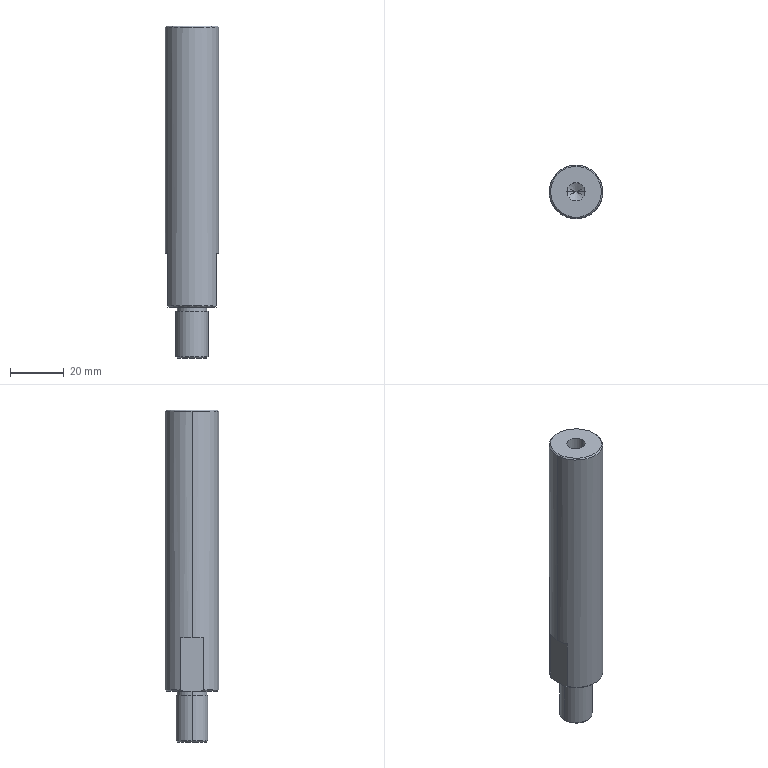Component | SolidWorks | SupportWheelAssembly-1_SupportWheelAxis-1 | 1 solid | 24 faces | box 20 x 20 x 124 mm | volume 34114 mm3 | cylinder 8 | cone 8 | plane 8 | commonest cylinder face diameters 6.8 x2 12 x2 11 x2 20 x2
build123d program:
from build123d import *

# Parameters (mm, degrees)
SKETCH1_R             = 10
BOSS_EXTRUDE1_DEPTH   = 52.5
CHAMFER1_SIZE         = 0.5
SKETCH4_W             = 7.858
SKETCH4_H             = 16.97
SKETCH4_W_2           = 6.894
SKETCH4_H_2           = 20.345
CUT_EXTRUDE1_DEPTH    = 20
SKETCH5_R             = 6
BOSS_EXTRUDE2_DEPTH   = 19
CHAMFER2_SIZE         = 0.5
SKETCH6_R             = 6
SKETCH6_R_2           = 5.5
CUT_EXTRUDE2_DEPTH    = 1.5
M8_TAPPED_HOLE1_D     = 6.8
M8_TAPPED_HOLE1_DEPTH = 19.75
M8_TAPPED_HOLE1_TIP   = 2.043


with BuildPart() as part:
    # Sketch1 → Boss-Extrude1 (new, symmetric)
    with BuildSketch(Plane.XY):
        Circle(SKETCH1_R)
    extrude(amount=BOSS_EXTRUDE1_DEPTH, both=True)

    # Chamfer1
    chamfer1_edges = [part.edges().sort_by_distance(p)[0] for p in [
        (-10, 0, -52.5),
        (-10, 0, 52.5),
    ]]
    chamfer(chamfer1_edges, length=CHAMFER1_SIZE)

    # Sketch4 → Cut-Extrude1 (cut)
    with BuildSketch(Plane(origin=(0, 0, -52.5), x_dir=(-1, 0, 0), z_dir=(0, 0, -1))):
        with Locations((-12.929, 0.3857)):
            Rectangle(SKETCH4_W, SKETCH4_H)
        with Locations((12.447, -0.916)):
            Rectangle(SKETCH4_W_2, SKETCH4_H_2)
    extrude(amount=-CUT_EXTRUDE1_DEPTH, mode=Mode.SUBTRACT)

    # Sketch5 → Boss-Extrude2 (add)
    with BuildSketch(Plane(origin=(0, 0, -52.5), x_dir=(-1, 0, 0), z_dir=(0, 0, -1))):
        with Locations(Location((0, 0, 0), (0, 0, 180))):
            Circle(SKETCH5_R)
    extrude(amount=BOSS_EXTRUDE2_DEPTH)

    # Chamfer2
    chamfer2_edges = [part.edges().sort_by_distance(p)[0] for p in [
        (-6, 0, -71.5),
    ]]
    chamfer(chamfer2_edges, length=CHAMFER2_SIZE)

    # Sketch6 → Cut-Extrude2 (cut)
    with BuildSketch(Plane(origin=(0, 0, -52.5), x_dir=(-1, 0, 0), z_dir=(0, 0, -1))):
        Circle(SKETCH6_R)
        Circle(SKETCH6_R_2, mode=Mode.SUBTRACT)
    extrude(amount=CUT_EXTRUDE2_DEPTH, mode=Mode.SUBTRACT)

    # M8 Tapped Hole1
    with Locations(Plane.XY.offset(52.5)):
        with Locations((0, 0)):
            Hole(M8_TAPPED_HOLE1_D / 2, depth=M8_TAPPED_HOLE1_DEPTH)
            with Locations((0, 0, -(M8_TAPPED_HOLE1_DEPTH + M8_TAPPED_HOLE1_TIP / 2))):  # 118° drill point
                Cone(0, M8_TAPPED_HOLE1_D / 2, M8_TAPPED_HOLE1_TIP, mode=Mode.SUBTRACT)


solid = part.part

# Placed as in the assembly
solid = solid.moved(Location((-187.007, -195.411, 567.5), (0, 0, 0)))
STEP:
#1=COLOUR_RGB('',0.7922,0.8196,0.9333);
#2=FILL_AREA_STYLE_COLOUR('',#1);
#3=FILL_AREA_STYLE('',(#2));
#4=SURFACE_STYLE_FILL_AREA(#3);
#5=SURFACE_SIDE_STYLE('',(#4));
#6=SURFACE_STYLE_USAGE(.BOTH.,#5);
#7=PRESENTATION_STYLE_ASSIGNMENT((#6));
#8=CARTESIAN_POINT('',(-7.496,-7.693,23.632));
#9=VERTEX_POINT('',#8);
#10=CARTESIAN_POINT('',(-7.229,-7.693,23.632));
#11=VERTEX_POINT('',#10);
#12=CARTESIAN_POINT('',(-7.362,-7.693,23.632));
#13=DIRECTION('',(0.,0.,1.));
#14=DIRECTION('',(1.,0.,0.));
#15=AXIS2_PLACEMENT_3D('',#12,#13,#14);
#16=CIRCLE('',#15,0.1339);
#17=EDGE_CURVE('',#9,#11,#16,.T.);
#18=ORIENTED_EDGE('',*,*,#17,.F.);
#19=CARTESIAN_POINT('',(-7.496,-7.693,24.409));
#20=VERTEX_POINT('',#19);
#21=CARTESIAN_POINT('',(-7.496,-7.693,24.409));
#22=DIRECTION('',(0.,0.,1.));
#23=VECTOR('',#22,39.37);
#24=LINE('',#21,#23);
#25=EDGE_CURVE('',#9,#20,#24,.T.);
#26=ORIENTED_EDGE('',*,*,#25,.T.);
#27=CARTESIAN_POINT('',(-7.229,-7.693,24.409));
#28=VERTEX_POINT('',#27);
#29=CARTESIAN_POINT('',(-7.362,-7.693,24.409));
#30=DIRECTION('',(0.,0.,1.));
#31=DIRECTION('',(1.,0.,0.));
#32=AXIS2_PLACEMENT_3D('',#29,#30,#31);
#33=CIRCLE('',#32,0.1339);
#34=EDGE_CURVE('',#20,#28,#33,.T.);
#35=ORIENTED_EDGE('',*,*,#34,.T.);
#36=CARTESIAN_POINT('',(-7.229,-7.693,24.409));
#37=DIRECTION('',(0.,0.,1.));
#38=VECTOR('',#37,39.37);
#39=LINE('',#36,#38);
#40=EDGE_CURVE('',#11,#28,#39,.T.);
#41=ORIENTED_EDGE('',*,*,#40,.F.);
#42=EDGE_LOOP('',(#18,#26,#35,#41));
#43=FACE_OUTER_BOUND('',#42,.T.);
#44=CARTESIAN_POINT('',(-7.362,-7.693,24.409));
#45=DIRECTION('',(0.,0.,1.));
#46=DIRECTION('',(1.,0.,0.));
#47=AXIS2_PLACEMENT_3D('',#44,#45,#46);
#48=CYLINDRICAL_SURFACE('',#47,0.1339);
#49=ADVANCED_FACE('',(#43),#48,.F.);
#50=CARTESIAN_POINT('',(-7.362,-7.693,23.551));
#51=VERTEX_POINT('',#50);
#52=CARTESIAN_POINT('',(-7.229,-7.693,23.632));
#53=DIRECTION('',(0.8572,0.,0.515));
#54=VECTOR('',#53,39.37);
#55=LINE('',#52,#54);
#56=EDGE_CURVE('',#51,#11,#55,.T.);
#57=ORIENTED_EDGE('',*,*,#56,.F.);
#58=CARTESIAN_POINT('',(-7.496,-7.693,23.632));
#59=DIRECTION('',(-0.8572,0.,0.515));
#60=VECTOR('',#59,39.37);
#61=LINE('',#58,#60);
#62=EDGE_CURVE('',#51,#9,#61,.T.);
#63=ORIENTED_EDGE('',*,*,#62,.T.);
#64=ORIENTED_EDGE('',*,*,#17,.T.);
#65=EDGE_LOOP('',(#57,#63,#64));
#66=FACE_OUTER_BOUND('',#65,.T.);
#67=CARTESIAN_POINT('',(-7.362,-7.693,23.632));
#68=DIRECTION('',(0.,0.,1.));
#69=DIRECTION('',(1.,0.,0.));
#70=AXIS2_PLACEMENT_3D('',#67,#68,#69);
#71=CONICAL_SURFACE('',#70,0.1339,1.03);
#72=ADVANCED_FACE('',(#66),#71,.F.);
#73=CARTESIAN_POINT('',(-7.126,-7.693,19.547));
#74=VERTEX_POINT('',#73);
#75=CARTESIAN_POINT('',(-7.599,-7.693,19.547));
#76=VERTEX_POINT('',#75);
#77=CARTESIAN_POINT('',(-7.362,-7.693,19.547));
#78=DIRECTION('',(0.,0.,1.));
#79=DIRECTION('',(-1.,0.,0.));
#80=AXIS2_PLACEMENT_3D('',#77,#78,#79);
#81=CIRCLE('',#80,0.2362);
#82=EDGE_CURVE('',#74,#76,#81,.T.);
#83=ORIENTED_EDGE('',*,*,#82,.T.);
#84=CARTESIAN_POINT('',(-7.599,-7.693,20.217));
#85=VERTEX_POINT('',#84);
#86=CARTESIAN_POINT('',(-7.599,-7.693,19.528));
#87=DIRECTION('',(0.,0.,1.));
#88=VECTOR('',#87,39.37);
#89=LINE('',#86,#88);
#90=EDGE_CURVE('',#76,#85,#89,.T.);
#91=ORIENTED_EDGE('',*,*,#90,.T.);
#92=CARTESIAN_POINT('',(-7.126,-7.693,20.217));
#93=VERTEX_POINT('',#92);
#94=CARTESIAN_POINT('',(-7.362,-7.693,20.217));
#95=DIRECTION('',(0.,0.,-1.));
#96=DIRECTION('',(-1.,0.,0.));
#97=AXIS2_PLACEMENT_3D('',#94,#95,#96);
#98=CIRCLE('',#97,0.2362);
#99=EDGE_CURVE('',#85,#93,#98,.T.);
#100=ORIENTED_EDGE('',*,*,#99,.T.);
#101=CARTESIAN_POINT('',(-7.126,-7.693,19.528));
#102=DIRECTION('',(0.,0.,1.));
#103=VECTOR('',#102,39.37);
#104=LINE('',#101,#103);
#105=EDGE_CURVE('',#74,#93,#104,.T.);
#106=ORIENTED_EDGE('',*,*,#105,.F.);
#107=EDGE_LOOP('',(#83,#91,#100,#106));
#108=FACE_OUTER_BOUND('',#107,.T.);
#109=CARTESIAN_POINT('',(-7.362,-7.693,19.528));
#110=DIRECTION('',(0.,0.,1.));
#111=DIRECTION('',(1.,0.,0.));
#112=AXIS2_PLACEMENT_3D('',#109,#110,#111);
#113=CYLINDRICAL_SURFACE('',#112,0.2362);
#114=ADVANCED_FACE('',(#108),#113,.T.);
#115=CARTESIAN_POINT('',(-7.579,-7.693,19.528));
#116=VERTEX_POINT('',#115);
#117=CARTESIAN_POINT('',(-7.146,-7.693,19.528));
#118=VERTEX_POINT('',#117);
#119=CARTESIAN_POINT('',(-7.362,-7.693,19.528));
#120=DIRECTION('',(0.,0.,-1.));
#121=DIRECTION('',(-1.,0.,0.));
#122=AXIS2_PLACEMENT_3D('',#119,#120,#121);
#123=CIRCLE('',#122,0.2165);
#124=EDGE_CURVE('',#116,#118,#123,.T.);
#125=ORIENTED_EDGE('',*,*,#124,.F.);
#126=CARTESIAN_POINT('',(-7.579,-7.693,19.528));
#127=DIRECTION('',(-0.7071,0.,0.7071));
#128=VECTOR('',#127,39.37);
#129=LINE('',#126,#128);
#130=EDGE_CURVE('',#116,#76,#129,.T.);
#131=ORIENTED_EDGE('',*,*,#130,.T.);
#132=ORIENTED_EDGE('',*,*,#82,.F.);
#133=CARTESIAN_POINT('',(-7.146,-7.693,19.528));
#134=DIRECTION('',(0.7071,0.,0.7071));
#135=VECTOR('',#134,39.37);
#136=LINE('',#133,#135);
#137=EDGE_CURVE('',#118,#74,#136,.T.);
#138=ORIENTED_EDGE('',*,*,#137,.F.);
#139=EDGE_LOOP('',(#125,#131,#132,#138));
#140=FACE_OUTER_BOUND('',#139,.T.);
#141=CARTESIAN_POINT('',(-7.362,-7.693,19.528));
#142=DIRECTION('',(0.,0.,1.));
#143=DIRECTION('',(1.,0.,0.));
#144=AXIS2_PLACEMENT_3D('',#141,#142,#143);
#145=CONICAL_SURFACE('',#144,0.2165,0.7854);
#146=ADVANCED_FACE('',(#140),#145,.T.);
#147=CARTESIAN_POINT('',(-7.579,-7.693,20.217));
#148=VERTEX_POINT('',#147);
#149=CARTESIAN_POINT('',(-7.146,-7.693,20.217));
#150=VERTEX_POINT('',#149);
#151=CARTESIAN_POINT('',(-7.362,-7.693,20.217));
#152=DIRECTION('',(0.,0.,-1.));
#153=DIRECTION('',(-1.,0.,0.));
#154=AXIS2_PLACEMENT_3D('',#151,#152,#153);
#155=CIRCLE('',#154,0.2165);
#156=EDGE_CURVE('',#148,#150,#155,.T.);
#157=ORIENTED_EDGE('',*,*,#156,.F.);
#158=CARTESIAN_POINT('',(-7.579,-7.693,20.276));
#159=VERTEX_POINT('',#158);
#160=CARTESIAN_POINT('',(-7.579,-7.693,20.217));
#161=DIRECTION('',(0.,0.,1.));
#162=VECTOR('',#161,39.37);
#163=LINE('',#160,#162);
#164=EDGE_CURVE('',#148,#159,#163,.T.);
#165=ORIENTED_EDGE('',*,*,#164,.T.);
#166=CARTESIAN_POINT('',(-7.146,-7.693,20.276));
#167=VERTEX_POINT('',#166);
#168=CARTESIAN_POINT('',(-7.362,-7.693,20.276));
#169=DIRECTION('',(0.,0.,-1.));
#170=DIRECTION('',(-1.,0.,0.));
#171=AXIS2_PLACEMENT_3D('',#168,#169,#170);
#172=CIRCLE('',#171,0.2165);
#173=EDGE_CURVE('',#159,#167,#172,.T.);
#174=ORIENTED_EDGE('',*,*,#173,.T.);
#175=CARTESIAN_POINT('',(-7.146,-7.693,20.217));
#176=DIRECTION('',(0.,0.,1.));
#177=VECTOR('',#176,39.37);
#178=LINE('',#175,#177);
#179=EDGE_CURVE('',#150,#167,#178,.T.);
#180=ORIENTED_EDGE('',*,*,#179,.F.);
#181=EDGE_LOOP('',(#157,#165,#174,#180));
#182=FACE_OUTER_BOUND('',#181,.T.);
#183=CARTESIAN_POINT('',(-7.362,-7.693,20.217));
#184=DIRECTION('',(0.,0.,1.));
#185=DIRECTION('',(1.,0.,0.));
#186=AXIS2_PLACEMENT_3D('',#183,#184,#185);
#187=CYLINDRICAL_SURFACE('',#186,0.2165);
#188=ADVANCED_FACE('',(#182),#187,.T.);
#189=CARTESIAN_POINT('',(-6.988,-7.693,24.409));
#190=VERTEX_POINT('',#189);
#191=CARTESIAN_POINT('',(-7.736,-7.693,24.409));
#192=VERTEX_POINT('',#191);
#193=CARTESIAN_POINT('',(-7.362,-7.693,24.409));
#194=DIRECTION('',(0.,0.,1.));
#195=DIRECTION('',(1.,0.,0.));
#196=AXIS2_PLACEMENT_3D('',#193,#194,#195);
#197=CIRCLE('',#196,0.374);
#198=EDGE_CURVE('',#190,#192,#197,.T.);
#199=ORIENTED_EDGE('',*,*,#198,.F.);
#200=CARTESIAN_POINT('',(-6.969,-7.693,24.39));
#201=VERTEX_POINT('',#200);
#202=CARTESIAN_POINT('',(-6.988,-7.693,24.409));
#203=DIRECTION('',(0.7071,0.,-0.7071));
#204=VECTOR('',#203,39.37);
#205=LINE('',#202,#204);
#206=EDGE_CURVE('',#190,#201,#205,.T.);
#207=ORIENTED_EDGE('',*,*,#206,.T.);
#208=CARTESIAN_POINT('',(-7.756,-7.693,24.39));
#209=VERTEX_POINT('',#208);
#210=CARTESIAN_POINT('',(-7.362,-7.693,24.39));
#211=DIRECTION('',(0.,0.,-1.));
#212=DIRECTION('',(1.,0.,0.));
#213=AXIS2_PLACEMENT_3D('',#210,#211,#212);
#214=CIRCLE('',#213,0.3937);
#215=EDGE_CURVE('',#209,#201,#214,.T.);
#216=ORIENTED_EDGE('',*,*,#215,.F.);
#217=CARTESIAN_POINT('',(-7.736,-7.693,24.409));
#218=DIRECTION('',(-0.7071,0.,-0.7071));
#219=VECTOR('',#218,39.37);
#220=LINE('',#217,#219);
#221=EDGE_CURVE('',#192,#209,#220,.T.);
#222=ORIENTED_EDGE('',*,*,#221,.F.);
#223=EDGE_LOOP('',(#199,#207,#216,#222));
#224=FACE_OUTER_BOUND('',#223,.T.);
#225=CARTESIAN_POINT('',(-7.362,-7.693,24.409));
#226=DIRECTION('',(0.,0.,-1.));
#227=DIRECTION('',(-1.,0.,0.));
#228=AXIS2_PLACEMENT_3D('',#225,#226,#227);
#229=CONICAL_SURFACE('',#228,0.374,0.7854);
#230=ADVANCED_FACE('',(#224),#229,.T.);
#231=ORIENTED_EDGE('',*,*,#215,.T.);
#232=CARTESIAN_POINT('',(-6.969,-7.693,21.063));
#233=VERTEX_POINT('',#232);
#234=CARTESIAN_POINT('',(-6.969,-7.693,24.409));
#235=DIRECTION('',(0.,0.,-1.));
#236=VECTOR('',#235,39.37);
#237=LINE('',#234,#236);
#238=EDGE_CURVE('',#201,#233,#237,.T.);
#239=ORIENTED_EDGE('',*,*,#238,.T.);
#240=CARTESIAN_POINT('',(-7.008,-7.522,21.063));
#241=VERTEX_POINT('',#240);
#242=CARTESIAN_POINT('',(-7.362,-7.693,21.063));
#243=DIRECTION('',(0.,0.,-1.));
#244=DIRECTION('',(-1.,0.,0.));
#245=AXIS2_PLACEMENT_3D('',#242,#243,#244);
#246=CIRCLE('',#245,0.3937);
#247=EDGE_CURVE('',#241,#233,#246,.T.);
#248=ORIENTED_EDGE('',*,*,#247,.F.);
#249=CARTESIAN_POINT('',(-7.008,-7.522,20.295));
#250=VERTEX_POINT('',#249);
#251=CARTESIAN_POINT('',(-7.008,-7.522,24.409));
#252=DIRECTION('',(0.,0.,-1.));
#253=VECTOR('',#252,39.37);
#254=LINE('',#251,#253);
#255=EDGE_CURVE('',#241,#250,#254,.T.);
#256=ORIENTED_EDGE('',*,*,#255,.T.);
#257=CARTESIAN_POINT('',(-7.717,-7.522,20.295));
#258=VERTEX_POINT('',#257);
#259=CARTESIAN_POINT('',(-7.362,-7.693,20.295));
#260=DIRECTION('',(0.,0.,1.));
#261=DIRECTION('',(1.,0.,0.));
#262=AXIS2_PLACEMENT_3D('',#259,#260,#261);
#263=CIRCLE('',#262,0.3937);
#264=EDGE_CURVE('',#250,#258,#263,.T.);
#265=ORIENTED_EDGE('',*,*,#264,.T.);
#266=CARTESIAN_POINT('',(-7.717,-7.522,21.063));
#267=VERTEX_POINT('',#266);
#268=CARTESIAN_POINT('',(-7.717,-7.522,24.409));
#269=DIRECTION('',(0.,0.,1.));
#270=VECTOR('',#269,39.37);
#271=LINE('',#268,#270);
#272=EDGE_CURVE('',#258,#267,#271,.T.);
#273=ORIENTED_EDGE('',*,*,#272,.T.);
#274=CARTESIAN_POINT('',(-7.756,-7.693,21.063));
#275=VERTEX_POINT('',#274);
#276=CARTESIAN_POINT('',(-7.362,-7.693,21.063));
#277=DIRECTION('',(0.,0.,1.));
#278=DIRECTION('',(1.,0.,0.));
#279=AXIS2_PLACEMENT_3D('',#276,#277,#278);
#280=CIRCLE('',#279,0.3937);
#281=EDGE_CURVE('',#267,#275,#280,.T.);
#282=ORIENTED_EDGE('',*,*,#281,.T.);
#283=CARTESIAN_POINT('',(-7.756,-7.693,24.409));
#284=DIRECTION('',(0.,0.,-1.));
#285=VECTOR('',#284,39.37);
#286=LINE('',#283,#285);
#287=EDGE_CURVE('',#209,#275,#286,.T.);
#288=ORIENTED_EDGE('',*,*,#287,.F.);
#289=EDGE_LOOP('',(#231,#239,#248,#256,#265,#273,#282,#288));
#290=FACE_OUTER_BOUND('',#289,.T.);
#291=CARTESIAN_POINT('',(-7.362,-7.693,24.409));
#292=DIRECTION('',(0.,0.,-1.));
#293=DIRECTION('',(-1.,0.,0.));
#294=AXIS2_PLACEMENT_3D('',#291,#292,#293);
#295=CYLINDRICAL_SURFACE('',#294,0.3937);
#296=ADVANCED_FACE('',(#290),#295,.T.);
#297=CARTESIAN_POINT('',(-7.717,-7.574,20.276));
#298=VERTEX_POINT('',#297);
#299=CARTESIAN_POINT('',(-7.717,-7.522,20.295));
#300=CARTESIAN_POINT('',(-7.717,-7.539,20.288));
#301=CARTESIAN_POINT('',(-7.717,-7.556,20.281));
#302=CARTESIAN_POINT('',(-7.717,-7.574,20.276));
#303=B_SPLINE_CURVE_WITH_KNOTS('',3,(#299,#300,#301,#302),.UNSPECIFIED.,.F.,.F.,(4,4),(0.01919,0.0206),.UNSPECIFIED.);
#304=EDGE_CURVE('',#258,#298,#303,.T.);
#305=ORIENTED_EDGE('',*,*,#304,.F.);
#306=ORIENTED_EDGE('',*,*,#264,.F.);
#307=CARTESIAN_POINT('',(-7.008,-7.574,20.276));
#308=VERTEX_POINT('',#307);
#309=CARTESIAN_POINT('',(-7.008,-7.574,20.276));
#310=CARTESIAN_POINT('',(-7.008,-7.556,20.281));
#311=CARTESIAN_POINT('',(-7.008,-7.539,20.288));
#312=CARTESIAN_POINT('',(-7.008,-7.522,20.295));
#313=B_SPLINE_CURVE_WITH_KNOTS('',3,(#309,#310,#311,#312),.UNSPECIFIED.,.F.,.F.,(4,4),(0.02475,0.02616),.UNSPECIFIED.);
#314=EDGE_CURVE('',#308,#250,#313,.T.);
#315=ORIENTED_EDGE('',*,*,#314,.F.);
#316=CARTESIAN_POINT('',(-7.362,-7.693,20.276));
#317=DIRECTION('',(0.,0.,-1.));
#318=DIRECTION('',(1.,0.,0.));
#319=AXIS2_PLACEMENT_3D('',#316,#317,#318);
#320=CIRCLE('',#319,0.374);
#321=EDGE_CURVE('',#298,#308,#320,.T.);
#322=ORIENTED_EDGE('',*,*,#321,.F.);
#323=EDGE_LOOP('',(#305,#306,#315,#322));
#324=FACE_OUTER_BOUND('',#323,.T.);
#325=CARTESIAN_POINT('',(-7.362,-7.693,20.295));
#326=DIRECTION('',(0.,0.,1.));
#327=DIRECTION('',(1.,0.,0.));
#328=AXIS2_PLACEMENT_3D('',#325,#326,#327);
#329=CONICAL_SURFACE('',#328,0.3937,0.7854);
#330=ADVANCED_FACE('',(#324),#329,.T.);
#331=ORIENTED_EDGE('',*,*,#238,.F.);
#332=CARTESIAN_POINT('',(-7.362,-7.693,24.39));
#333=DIRECTION('',(0.,0.,-1.));
#334=DIRECTION('',(1.,0.,0.));
#335=AXIS2_PLACEMENT_3D('',#332,#333,#334);
#336=CIRCLE('',#335,0.3937);
#337=EDGE_CURVE('',#201,#209,#336,.T.);
#338=ORIENTED_EDGE('',*,*,#337,.T.);
#339=ORIENTED_EDGE('',*,*,#287,.T.);
#340=CARTESIAN_POINT('',(-7.717,-7.865,21.063));
#341=VERTEX_POINT('',#340);
#342=CARTESIAN_POINT('',(-7.362,-7.693,21.063));
#343=DIRECTION('',(0.,0.,1.));
#344=DIRECTION('',(1.,0.,0.));
#345=AXIS2_PLACEMENT_3D('',#342,#343,#344);
#346=CIRCLE('',#345,0.3937);
#347=EDGE_CURVE('',#275,#341,#346,.T.);
#348=ORIENTED_EDGE('',*,*,#347,.T.);
#349=CARTESIAN_POINT('',(-7.717,-7.865,20.295));
#350=VERTEX_POINT('',#349);
#351=CARTESIAN_POINT('',(-7.717,-7.865,24.409));
#352=DIRECTION('',(0.,0.,-1.));
#353=VECTOR('',#352,39.37);
#354=LINE('',#351,#353);
#355=EDGE_CURVE('',#341,#350,#354,.T.);
#356=ORIENTED_EDGE('',*,*,#355,.T.);
#357=CARTESIAN_POINT('',(-7.008,-7.865,20.295));
#358=VERTEX_POINT('',#357);
#359=CARTESIAN_POINT('',(-7.362,-7.693,20.295));
#360=DIRECTION('',(0.,0.,1.));
#361=DIRECTION('',(1.,0.,0.));
#362=AXIS2_PLACEMENT_3D('',#359,#360,#361);
#363=CIRCLE('',#362,0.3937);
#364=EDGE_CURVE('',#350,#358,#363,.T.);
#365=ORIENTED_EDGE('',*,*,#364,.T.);
#366=CARTESIAN_POINT('',(-7.008,-7.865,21.063));
#367=VERTEX_POINT('',#366);
#368=CARTESIAN_POINT('',(-7.008,-7.865,24.409));
#369=DIRECTION('',(0.,0.,1.));
#370=VECTOR('',#369,39.37);
#371=LINE('',#368,#370);
#372=EDGE_CURVE('',#358,#367,#371,.T.);
#373=ORIENTED_EDGE('',*,*,#372,.T.);
#374=CARTESIAN_POINT('',(-7.362,-7.693,21.063));
#375=DIRECTION('',(0.,0.,-1.));
#376=DIRECTION('',(-1.,0.,0.));
#377=AXIS2_PLACEMENT_3D('',#374,#375,#376);
#378=CIRCLE('',#377,0.3937);
#379=EDGE_CURVE('',#233,#367,#378,.T.);
#380=ORIENTED_EDGE('',*,*,#379,.F.);
#381=EDGE_LOOP('',(#331,#338,#339,#348,#356,#365,#373,#380));
#382=FACE_OUTER_BOUND('',#381,.T.);
#383=CARTESIAN_POINT('',(-7.362,-7.693,24.409));
#384=DIRECTION('',(0.,0.,-1.));
#385=DIRECTION('',(-1.,0.,0.));
#386=AXIS2_PLACEMENT_3D('',#383,#384,#385);
#387=CYLINDRICAL_SURFACE('',#386,0.3937);
#388=ADVANCED_FACE('',(#382),#387,.T.);
#389=CARTESIAN_POINT('',(-7.362,-7.693,24.409));
#390=DIRECTION('',(0.,0.,1.));
#391=DIRECTION('',(1.,0.,0.));
#392=AXIS2_PLACEMENT_3D('',#389,#390,#391);
#393=CIRCLE('',#392,0.1339);
#394=EDGE_CURVE('',#28,#20,#393,.T.);
#395=ORIENTED_EDGE('',*,*,#394,.F.);
#396=ORIENTED_EDGE('',*,*,#34,.F.);
#397=EDGE_LOOP('',(#395,#396));
#398=FACE_BOUND('',#397,.T.);
#399=CARTESIAN_POINT('',(-7.362,-7.693,24.409));
#400=DIRECTION('',(0.,0.,1.));
#401=DIRECTION('',(1.,0.,0.));
#402=AXIS2_PLACEMENT_3D('',#399,#400,#401);
#403=CIRCLE('',#402,0.374);
#404=EDGE_CURVE('',#192,#190,#403,.T.);
#405=ORIENTED_EDGE('',*,*,#404,.T.);
#406=ORIENTED_EDGE('',*,*,#198,.T.);
#407=EDGE_LOOP('',(#405,#406));
#408=FACE_OUTER_BOUND('',#407,.T.);
#409=CARTESIAN_POINT('',(-7.362,-7.693,24.409));
#410=DIRECTION('',(0.,0.,1.));
#411=DIRECTION('',(1.,0.,0.));
#412=AXIS2_PLACEMENT_3D('',#409,#410,#411);
#413=PLANE('',#412);
#414=ADVANCED_FACE('',(#398,#408),#413,.T.);
#415=CARTESIAN_POINT('',(-7.008,-7.813,20.276));
#416=VERTEX_POINT('',#415);
#417=CARTESIAN_POINT('',(-7.717,-7.813,20.276));
#418=VERTEX_POINT('',#417);
#419=CARTESIAN_POINT('',(-7.362,-7.693,20.276));
#420=DIRECTION('',(0.,0.,-1.));
#421=DIRECTION('',(1.,0.,0.));
#422=AXIS2_PLACEMENT_3D('',#419,#420,#421);
#423=CIRCLE('',#422,0.374);
#424=EDGE_CURVE('',#416,#418,#423,.T.);
#425=ORIENTED_EDGE('',*,*,#424,.T.);
#426=CARTESIAN_POINT('',(-7.717,-7.329,20.276));
#427=DIRECTION('',(-0.,-1.,0.));
#428=VECTOR('',#427,39.37);
#429=LINE('',#426,#428);
#430=EDGE_CURVE('',#298,#418,#429,.T.);
#431=ORIENTED_EDGE('',*,*,#430,.F.);
#432=ORIENTED_EDGE('',*,*,#321,.T.);
#433=CARTESIAN_POINT('',(-7.008,-7.344,20.276));
#434=DIRECTION('',(0.,1.,0.));
#435=VECTOR('',#434,39.37);
#436=LINE('',#433,#435);
#437=EDGE_CURVE('',#416,#308,#436,.T.);
#438=ORIENTED_EDGE('',*,*,#437,.F.);
#439=EDGE_LOOP('',(#425,#431,#432,#438));
#440=FACE_OUTER_BOUND('',#439,.T.);
#441=CARTESIAN_POINT('',(-7.362,-7.693,20.276));
#442=DIRECTION('',(0.,0.,-1.));
#443=DIRECTION('',(-1.,0.,0.));
#444=AXIS2_PLACEMENT_3D('',#441,#442,#443);
#445=CIRCLE('',#444,0.2165);
#446=EDGE_CURVE('',#167,#159,#445,.T.);
#447=ORIENTED_EDGE('',*,*,#446,.F.);
#448=ORIENTED_EDGE('',*,*,#173,.F.);
#449=EDGE_LOOP('',(#447,#448));
#450=FACE_BOUND('',#449,.T.);
#451=CARTESIAN_POINT('',(-7.362,-7.693,20.276));
#452=DIRECTION('',(0.,0.,1.));
#453=DIRECTION('',(1.,0.,0.));
#454=AXIS2_PLACEMENT_3D('',#451,#452,#453);
#455=PLANE('',#454);
#456=ADVANCED_FACE('',(#440,#450),#455,.F.);
#457=ORIENTED_EDGE('',*,*,#206,.F.);
#458=ORIENTED_EDGE('',*,*,#404,.F.);
#459=ORIENTED_EDGE('',*,*,#221,.T.);
#460=ORIENTED_EDGE('',*,*,#337,.F.);
#461=EDGE_LOOP('',(#457,#458,#459,#460));
#462=FACE_OUTER_BOUND('',#461,.T.);
#463=CARTESIAN_POINT('',(-7.362,-7.693,24.409));
#464=DIRECTION('',(0.,0.,-1.));
#465=DIRECTION('',(-1.,0.,0.));
#466=AXIS2_PLACEMENT_3D('',#463,#464,#465);
#467=CONICAL_SURFACE('',#466,0.374,0.7854);
#468=ADVANCED_FACE('',(#462),#467,.T.);
#469=CARTESIAN_POINT('',(-7.717,-7.813,20.276));
#470=CARTESIAN_POINT('',(-7.717,-7.831,20.281));
#471=CARTESIAN_POINT('',(-7.717,-7.848,20.288));
#472=CARTESIAN_POINT('',(-7.717,-7.865,20.295));
#473=B_SPLINE_CURVE_WITH_KNOTS('',3,(#469,#470,#471,#472),.UNSPECIFIED.,.F.,.F.,(4,4),(0.02679,0.02819),.UNSPECIFIED.);
#474=EDGE_CURVE('',#418,#350,#473,.T.);
#475=ORIENTED_EDGE('',*,*,#474,.F.);
#476=ORIENTED_EDGE('',*,*,#424,.F.);
#477=CARTESIAN_POINT('',(-7.008,-7.865,20.295));
#478=CARTESIAN_POINT('',(-7.008,-7.848,20.288));
#479=CARTESIAN_POINT('',(-7.008,-7.831,20.281));
#480=CARTESIAN_POINT('',(-7.008,-7.813,20.276));
#481=B_SPLINE_CURVE_WITH_KNOTS('',3,(#477,#478,#479,#480),.UNSPECIFIED.,.F.,.F.,(4,4),(0.01714,0.01855),.UNSPECIFIED.);
#482=EDGE_CURVE('',#358,#416,#481,.T.);
#483=ORIENTED_EDGE('',*,*,#482,.F.);
#484=ORIENTED_EDGE('',*,*,#364,.F.);
#485=EDGE_LOOP('',(#475,#476,#483,#484));
#486=FACE_OUTER_BOUND('',#485,.T.);
#487=CARTESIAN_POINT('',(-7.362,-7.693,20.295));
#488=DIRECTION('',(0.,0.,1.));
#489=DIRECTION('',(1.,0.,0.));
#490=AXIS2_PLACEMENT_3D('',#487,#488,#489);
#491=CONICAL_SURFACE('',#490,0.3937,0.7854);
#492=ADVANCED_FACE('',(#486),#491,.T.);
#493=ORIENTED_EDGE('',*,*,#247,.T.);
#494=ORIENTED_EDGE('',*,*,#379,.T.);
#495=CARTESIAN_POINT('',(-7.008,-7.344,21.063));
#496=DIRECTION('',(0.,1.,0.));
#497=VECTOR('',#496,39.37);
#498=LINE('',#495,#497);
#499=EDGE_CURVE('',#367,#241,#498,.T.);
#500=ORIENTED_EDGE('',*,*,#499,.T.);
#501=EDGE_LOOP('',(#493,#494,#500));
#502=FACE_OUTER_BOUND('',#501,.T.);
#503=CARTESIAN_POINT('',(-7.362,-7.693,21.063));
#504=DIRECTION('',(0.,0.,-1.));
#505=DIRECTION('',(-1.,0.,0.));
#506=AXIS2_PLACEMENT_3D('',#503,#504,#505);
#507=PLANE('',#506);
#508=ADVANCED_FACE('',(#502),#507,.T.);
#509=ORIENTED_EDGE('',*,*,#482,.T.);
#510=ORIENTED_EDGE('',*,*,#437,.T.);
#511=ORIENTED_EDGE('',*,*,#314,.T.);
#512=ORIENTED_EDGE('',*,*,#255,.F.);
#513=ORIENTED_EDGE('',*,*,#499,.F.);
#514=ORIENTED_EDGE('',*,*,#372,.F.);
#515=EDGE_LOOP('',(#509,#510,#511,#512,#513,#514));
#516=FACE_OUTER_BOUND('',#515,.T.);
#517=CARTESIAN_POINT('',(-7.008,-7.344,21.063));
#518=DIRECTION('',(-1.,0.,0.));
#519=DIRECTION('',(-0.,-1.,0.));
#520=AXIS2_PLACEMENT_3D('',#517,#518,#519);
#521=PLANE('',#520);
#522=ADVANCED_FACE('',(#516),#521,.F.);
#523=CARTESIAN_POINT('',(-7.717,-7.329,21.063));
#524=DIRECTION('',(-0.,-1.,0.));
#525=VECTOR('',#524,39.37);
#526=LINE('',#523,#525);
#527=EDGE_CURVE('',#267,#341,#526,.T.);
#528=ORIENTED_EDGE('',*,*,#527,.T.);
#529=ORIENTED_EDGE('',*,*,#347,.F.);
#530=ORIENTED_EDGE('',*,*,#281,.F.);
#531=EDGE_LOOP('',(#528,#529,#530));
#532=FACE_OUTER_BOUND('',#531,.T.);
#533=CARTESIAN_POINT('',(-7.362,-7.693,21.063));
#534=DIRECTION('',(0.,0.,1.));
#535=DIRECTION('',(1.,0.,0.));
#536=AXIS2_PLACEMENT_3D('',#533,#534,#535);
#537=PLANE('',#536);
#538=ADVANCED_FACE('',(#532),#537,.F.);
#539=ORIENTED_EDGE('',*,*,#304,.T.);
#540=ORIENTED_EDGE('',*,*,#430,.T.);
#541=ORIENTED_EDGE('',*,*,#474,.T.);
#542=ORIENTED_EDGE('',*,*,#355,.F.);
#543=ORIENTED_EDGE('',*,*,#527,.F.);
#544=ORIENTED_EDGE('',*,*,#272,.F.);
#545=EDGE_LOOP('',(#539,#540,#541,#542,#543,#544));
#546=FACE_OUTER_BOUND('',#545,.T.);
#547=CARTESIAN_POINT('',(-7.717,-7.329,21.063));
#548=DIRECTION('',(1.,-0.,0.));
#549=DIRECTION('',(0.,1.,0.));
#550=AXIS2_PLACEMENT_3D('',#547,#548,#549);
#551=PLANE('',#550);
#552=ADVANCED_FACE('',(#546),#551,.F.);
#553=CARTESIAN_POINT('',(-7.362,-7.693,20.217));
#554=DIRECTION('',(0.,0.,-1.));
#555=DIRECTION('',(-1.,0.,0.));
#556=AXIS2_PLACEMENT_3D('',#553,#554,#555);
#557=CIRCLE('',#556,0.2362);
#558=EDGE_CURVE('',#93,#85,#557,.T.);
#559=ORIENTED_EDGE('',*,*,#558,.F.);
#560=ORIENTED_EDGE('',*,*,#99,.F.);
#561=EDGE_LOOP('',(#559,#560));
#562=FACE_OUTER_BOUND('',#561,.T.);
#563=CARTESIAN_POINT('',(-7.362,-7.693,20.217));
#564=DIRECTION('',(0.,0.,-1.));
#565=DIRECTION('',(-1.,0.,0.));
#566=AXIS2_PLACEMENT_3D('',#563,#564,#565);
#567=CIRCLE('',#566,0.2165);
#568=EDGE_CURVE('',#150,#148,#567,.T.);
#569=ORIENTED_EDGE('',*,*,#568,.T.);
#570=ORIENTED_EDGE('',*,*,#156,.T.);
#571=EDGE_LOOP('',(#569,#570));
#572=FACE_BOUND('',#571,.T.);
#573=CARTESIAN_POINT('',(-7.362,-7.693,20.217));
#574=DIRECTION('',(0.,0.,-1.));
#575=DIRECTION('',(-1.,0.,0.));
#576=AXIS2_PLACEMENT_3D('',#573,#574,#575);
#577=PLANE('',#576);
#578=ADVANCED_FACE('',(#562,#572),#577,.F.);
#579=ORIENTED_EDGE('',*,*,#164,.F.);
#580=ORIENTED_EDGE('',*,*,#568,.F.);
#581=ORIENTED_EDGE('',*,*,#179,.T.);
#582=ORIENTED_EDGE('',*,*,#446,.T.);
#583=EDGE_LOOP('',(#579,#580,#581,#582));
#584=FACE_OUTER_BOUND('',#583,.T.);
#585=CARTESIAN_POINT('',(-7.362,-7.693,20.217));
#586=DIRECTION('',(0.,0.,1.));
#587=DIRECTION('',(1.,0.,0.));
#588=AXIS2_PLACEMENT_3D('',#585,#586,#587);
#589=CYLINDRICAL_SURFACE('',#588,0.2165);
#590=ADVANCED_FACE('',(#584),#589,.T.);
#591=CARTESIAN_POINT('',(-7.362,-7.693,19.528));
#592=DIRECTION('',(0.,0.,-1.));
#593=DIRECTION('',(-1.,0.,0.));
#594=AXIS2_PLACEMENT_3D('',#591,#592,#593);
#595=CIRCLE('',#594,0.2165);
#596=EDGE_CURVE('',#118,#116,#595,.T.);
#597=ORIENTED_EDGE('',*,*,#596,.T.);
#598=ORIENTED_EDGE('',*,*,#124,.T.);
#599=EDGE_LOOP('',(#597,#598));
#600=FACE_OUTER_BOUND('',#599,.T.);
#601=CARTESIAN_POINT('',(-7.362,-7.693,19.528));
#602=DIRECTION('',(0.,0.,-1.));
#603=DIRECTION('',(-1.,0.,0.));
#604=AXIS2_PLACEMENT_3D('',#601,#602,#603);
#605=PLANE('',#604);
#606=ADVANCED_FACE('',(#600),#605,.T.);
#607=ORIENTED_EDGE('',*,*,#130,.F.);
#608=ORIENTED_EDGE('',*,*,#596,.F.);
#609=ORIENTED_EDGE('',*,*,#137,.T.);
#610=CARTESIAN_POINT('',(-7.362,-7.693,19.547));
#611=DIRECTION('',(0.,0.,1.));
#612=DIRECTION('',(-1.,0.,0.));
#613=AXIS2_PLACEMENT_3D('',#610,#611,#612);
#614=CIRCLE('',#613,0.2362);
#615=EDGE_CURVE('',#76,#74,#614,.T.);
#616=ORIENTED_EDGE('',*,*,#615,.F.);
#617=EDGE_LOOP('',(#607,#608,#609,#616));
#618=FACE_OUTER_BOUND('',#617,.T.);
#619=CARTESIAN_POINT('',(-7.362,-7.693,19.528));
#620=DIRECTION('',(0.,0.,1.));
#621=DIRECTION('',(1.,0.,0.));
#622=AXIS2_PLACEMENT_3D('',#619,#620,#621);
#623=CONICAL_SURFACE('',#622,0.2165,0.7854);
#624=ADVANCED_FACE('',(#618),#623,.T.);
#625=ORIENTED_EDGE('',*,*,#90,.F.);
#626=ORIENTED_EDGE('',*,*,#615,.T.);
#627=ORIENTED_EDGE('',*,*,#105,.T.);
#628=ORIENTED_EDGE('',*,*,#558,.T.);
#629=EDGE_LOOP('',(#625,#626,#627,#628));
#630=FACE_OUTER_BOUND('',#629,.T.);
#631=CARTESIAN_POINT('',(-7.362,-7.693,19.528));
#632=DIRECTION('',(0.,0.,1.));
#633=DIRECTION('',(1.,0.,0.));
#634=AXIS2_PLACEMENT_3D('',#631,#632,#633);
#635=CYLINDRICAL_SURFACE('',#634,0.2362);
#636=ADVANCED_FACE('',(#630),#635,.T.);
#637=ORIENTED_EDGE('',*,*,#62,.F.);
#638=ORIENTED_EDGE('',*,*,#56,.T.);
#639=CARTESIAN_POINT('',(-7.362,-7.693,23.632));
#640=DIRECTION('',(0.,0.,1.));
#641=DIRECTION('',(1.,0.,0.));
#642=AXIS2_PLACEMENT_3D('',#639,#640,#641);
#643=CIRCLE('',#642,0.1339);
#644=EDGE_CURVE('',#11,#9,#643,.T.);
#645=ORIENTED_EDGE('',*,*,#644,.T.);
#646=EDGE_LOOP('',(#637,#638,#645));
#647=FACE_OUTER_BOUND('',#646,.T.);
#648=CARTESIAN_POINT('',(-7.362,-7.693,23.632));
#649=DIRECTION('',(0.,0.,1.));
#650=DIRECTION('',(1.,0.,0.));
#651=AXIS2_PLACEMENT_3D('',#648,#649,#650);
#652=CONICAL_SURFACE('',#651,0.1339,1.03);
#653=ADVANCED_FACE('',(#647),#652,.F.);
#654=ORIENTED_EDGE('',*,*,#25,.F.);
#655=ORIENTED_EDGE('',*,*,#644,.F.);
#656=ORIENTED_EDGE('',*,*,#40,.T.);
#657=ORIENTED_EDGE('',*,*,#394,.T.);
#658=EDGE_LOOP('',(#654,#655,#656,#657));
#659=FACE_OUTER_BOUND('',#658,.T.);
#660=CARTESIAN_POINT('',(-7.362,-7.693,24.409));
#661=DIRECTION('',(0.,0.,1.));
#662=DIRECTION('',(1.,0.,0.));
#663=AXIS2_PLACEMENT_3D('',#660,#661,#662);
#664=CYLINDRICAL_SURFACE('',#663,0.1339);
#665=ADVANCED_FACE('',(#659),#664,.F.);
#666=CLOSED_SHELL('',(#49,#72,#114,#146,#188,#230,#296,#330,#388,#414,#456,#468,#492,#508,#522,#538,#552,#578,#590,#606,#624,#636,#653,#665));
#667=MANIFOLD_SOLID_BREP('',#666);
#668=STYLED_ITEM('',(#7),#667);
#669=PRESENTATION_LAYER_ASSIGNMENT('','',(#668));
#670=(LENGTH_UNIT()NAMED_UNIT(*)SI_UNIT($,.METRE.));
#671=LENGTH_MEASURE_WITH_UNIT(LENGTH_MEASURE(0.0254),#670);
#672=DIMENSIONAL_EXPONENTS(1.,0.,0.,0.,0.,0.,0.);
#673=(CONVERSION_BASED_UNIT('',#671)LENGTH_UNIT()NAMED_UNIT(#672));
#674=UNCERTAINTY_MEASURE_WITH_UNIT(LENGTH_MEASURE(0.00001),#673,'','');
#675=(NAMED_UNIT(*)PLANE_ANGLE_UNIT()SI_UNIT($,.RADIAN.));
#676=(NAMED_UNIT(*)SI_UNIT($,.STERADIAN.)SOLID_ANGLE_UNIT());
#677=(GEOMETRIC_REPRESENTATION_CONTEXT(3)GLOBAL_UNCERTAINTY_ASSIGNED_CONTEXT((#674))GLOBAL_UNIT_ASSIGNED_CONTEXT((#673,#675,#676))REPRESENTATION_CONTEXT('',''));
#678=MECHANICAL_DESIGN_GEOMETRIC_PRESENTATION_REPRESENTATION('',(#668),#677);
#679=CARTESIAN_POINT('',(0.,0.,0.));
#680=DIRECTION('',(0.,0.,1.));
#681=DIRECTION('',(1.,0.,0.));
#682=AXIS2_PLACEMENT_3D('',#679,#680,#681);
#683=(LENGTH_UNIT()NAMED_UNIT(*)SI_UNIT($,.METRE.));
#684=LENGTH_MEASURE_WITH_UNIT(LENGTH_MEASURE(0.0254),#683);
#685=DIMENSIONAL_EXPONENTS(1.,0.,0.,0.,0.,0.,0.);
#686=(CONVERSION_BASED_UNIT('',#684)LENGTH_UNIT()NAMED_UNIT(#685));
#687=UNCERTAINTY_MEASURE_WITH_UNIT(LENGTH_MEASURE(0.00001),#686,'','');
#688=(NAMED_UNIT(*)PLANE_ANGLE_UNIT()SI_UNIT($,.RADIAN.));
#689=(NAMED_UNIT(*)SI_UNIT($,.STERADIAN.)SOLID_ANGLE_UNIT());
#690=(GEOMETRIC_REPRESENTATION_CONTEXT(3)GLOBAL_UNCERTAINTY_ASSIGNED_CONTEXT((#687))GLOBAL_UNIT_ASSIGNED_CONTEXT((#686,#688,#689))REPRESENTATION_CONTEXT('',''));
#691=ADVANCED_BREP_SHAPE_REPRESENTATION('',(#667,#682),#690);